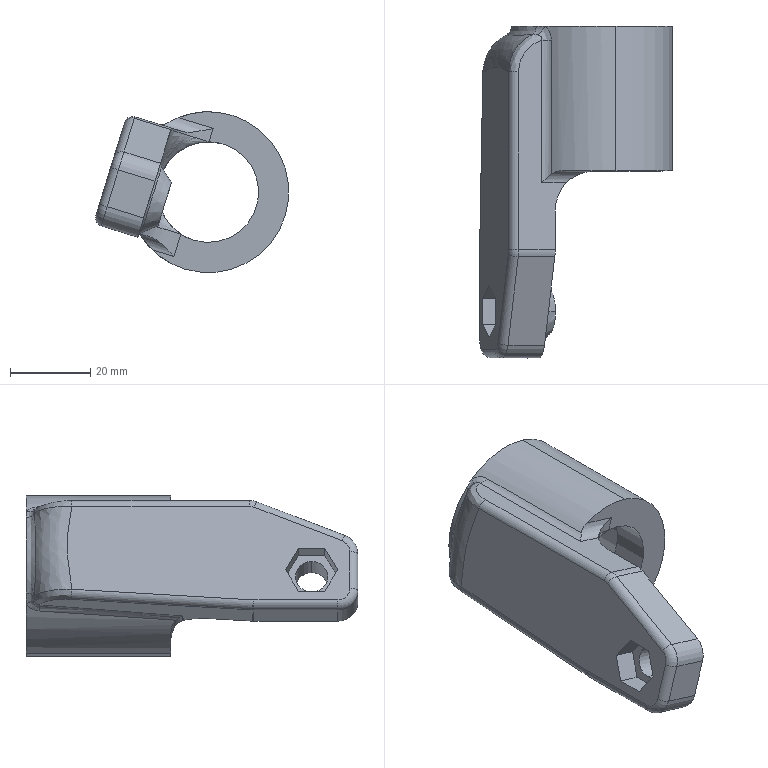Component | SolidWorks | DriveDevice-1_GuideWheelBracket-1 | 1 solid | 66 faces | volume 33276 mm3 | cylinder 28 | plane 20 | spline 10 | torus 6 | cone 2 | commonest cylinder face diameters 4 x5 6 x4 35 x4 10 x4 40 x3 25 x2 37 x2 8 x2